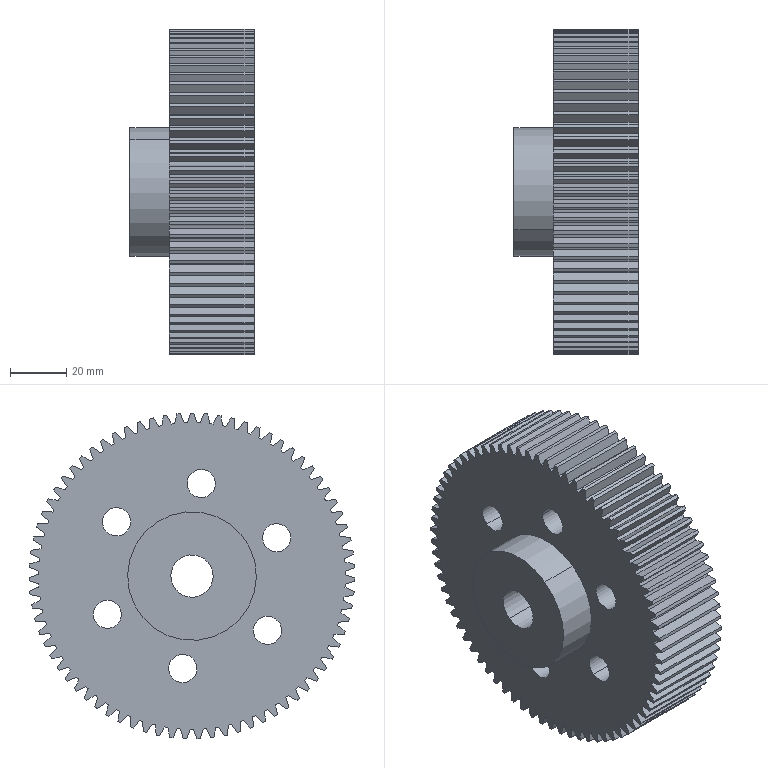Component | SolidWorks | ReducerLargeGear-4 | 1 solid | 341 faces | volume 291925 mm3 | cylinder 181 | spline 150 | plane 10 | commonest cylinder face diameters 115.5 x76 108.75 x75 15 x14 10 x12 45.636 x2 28.138 x2